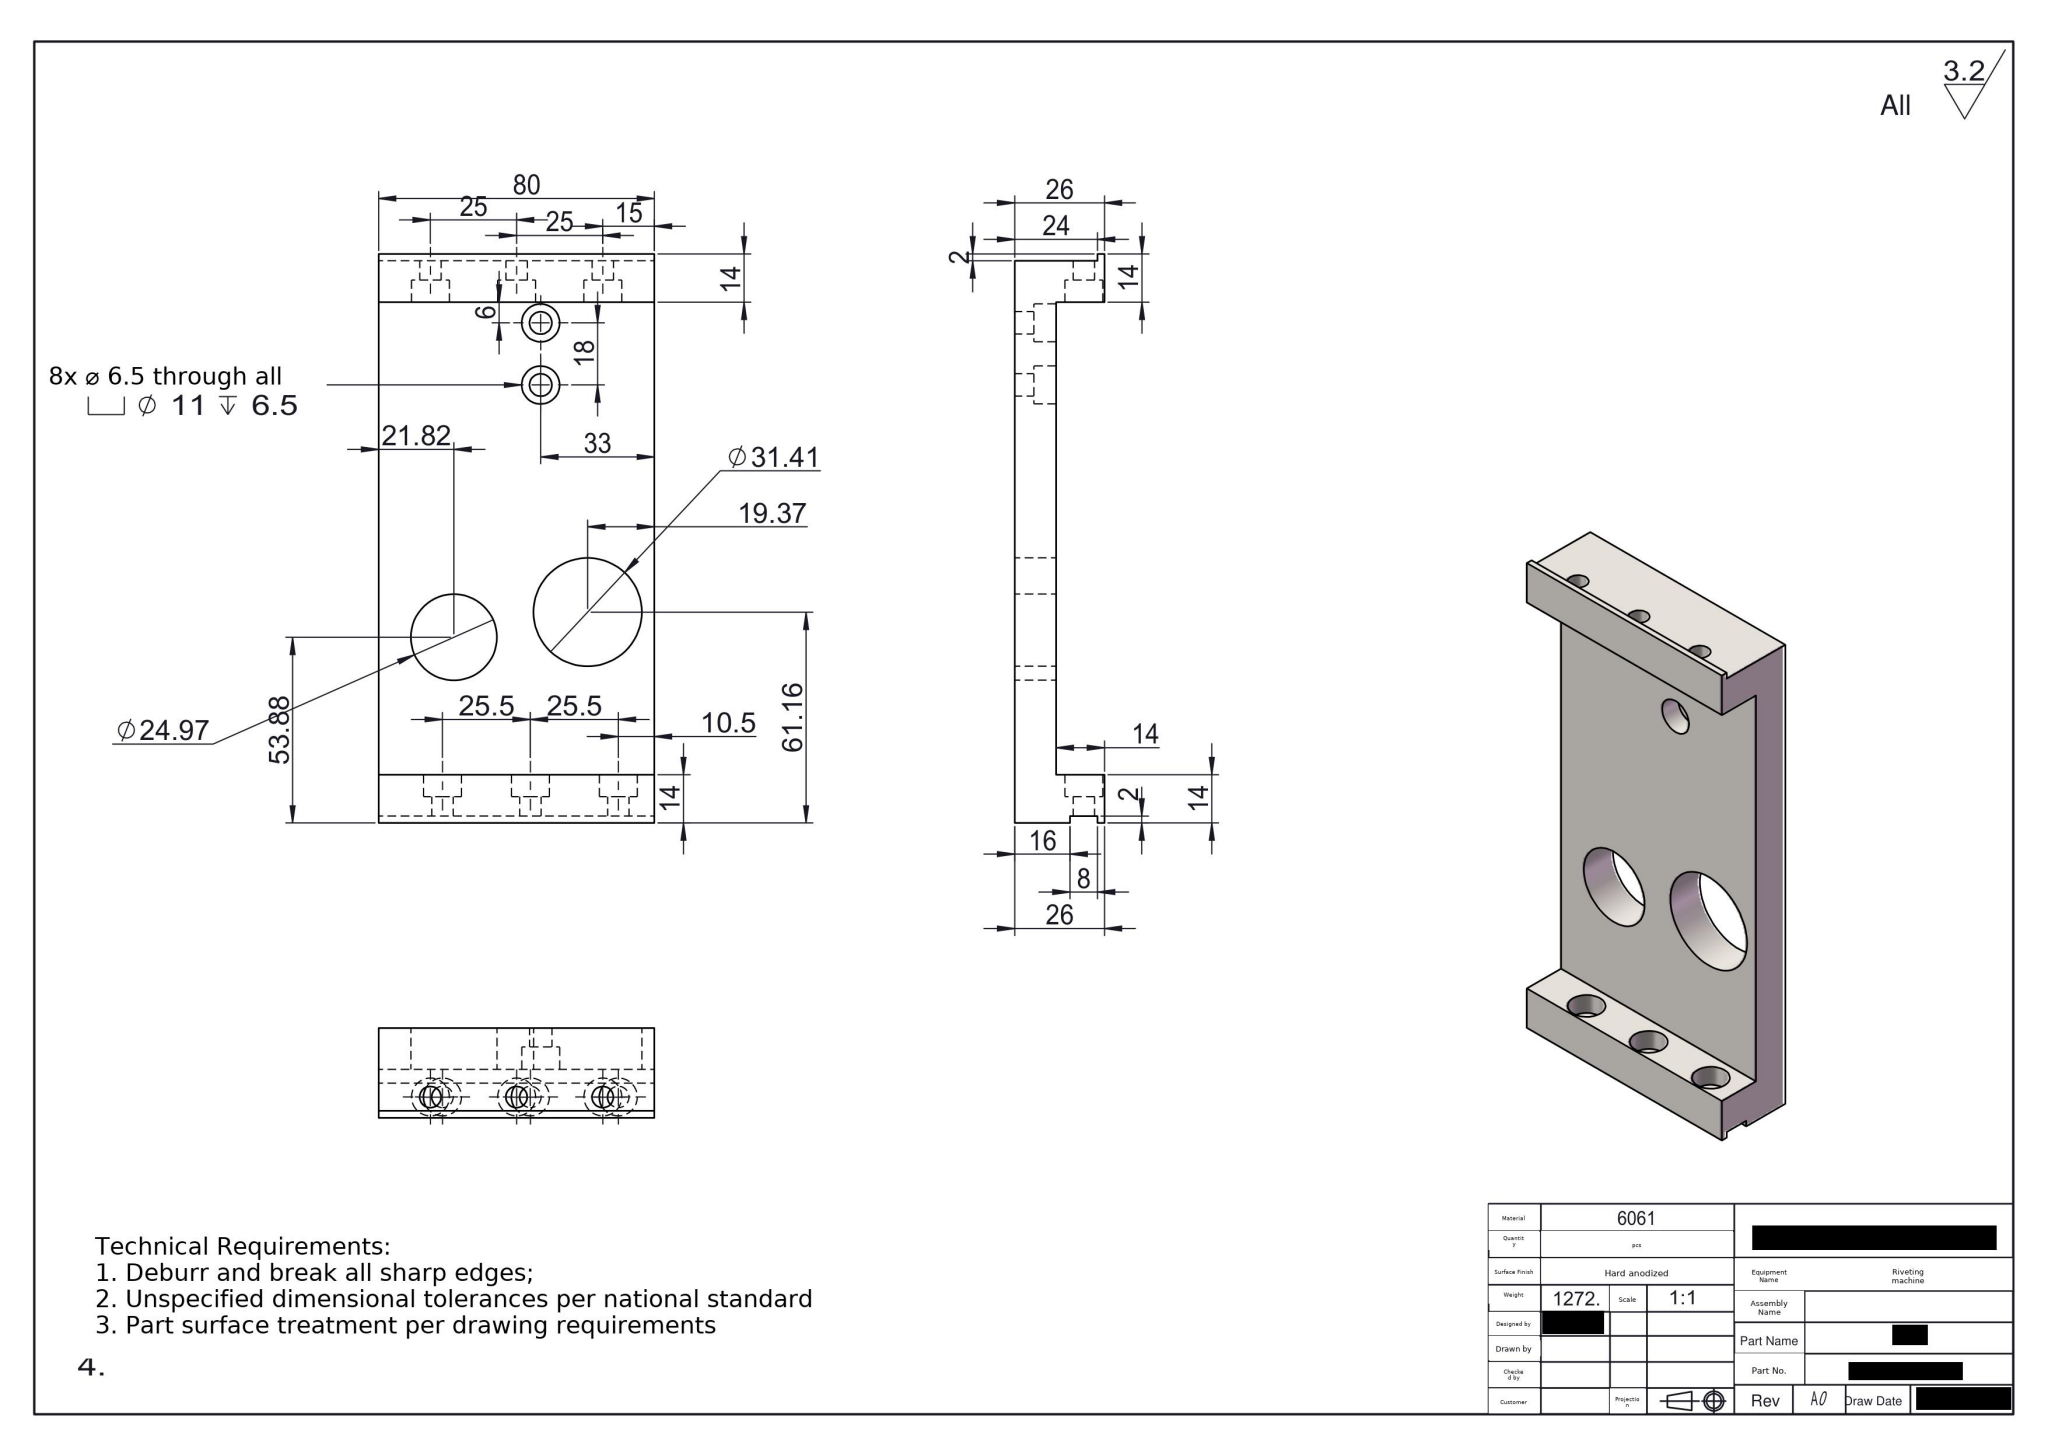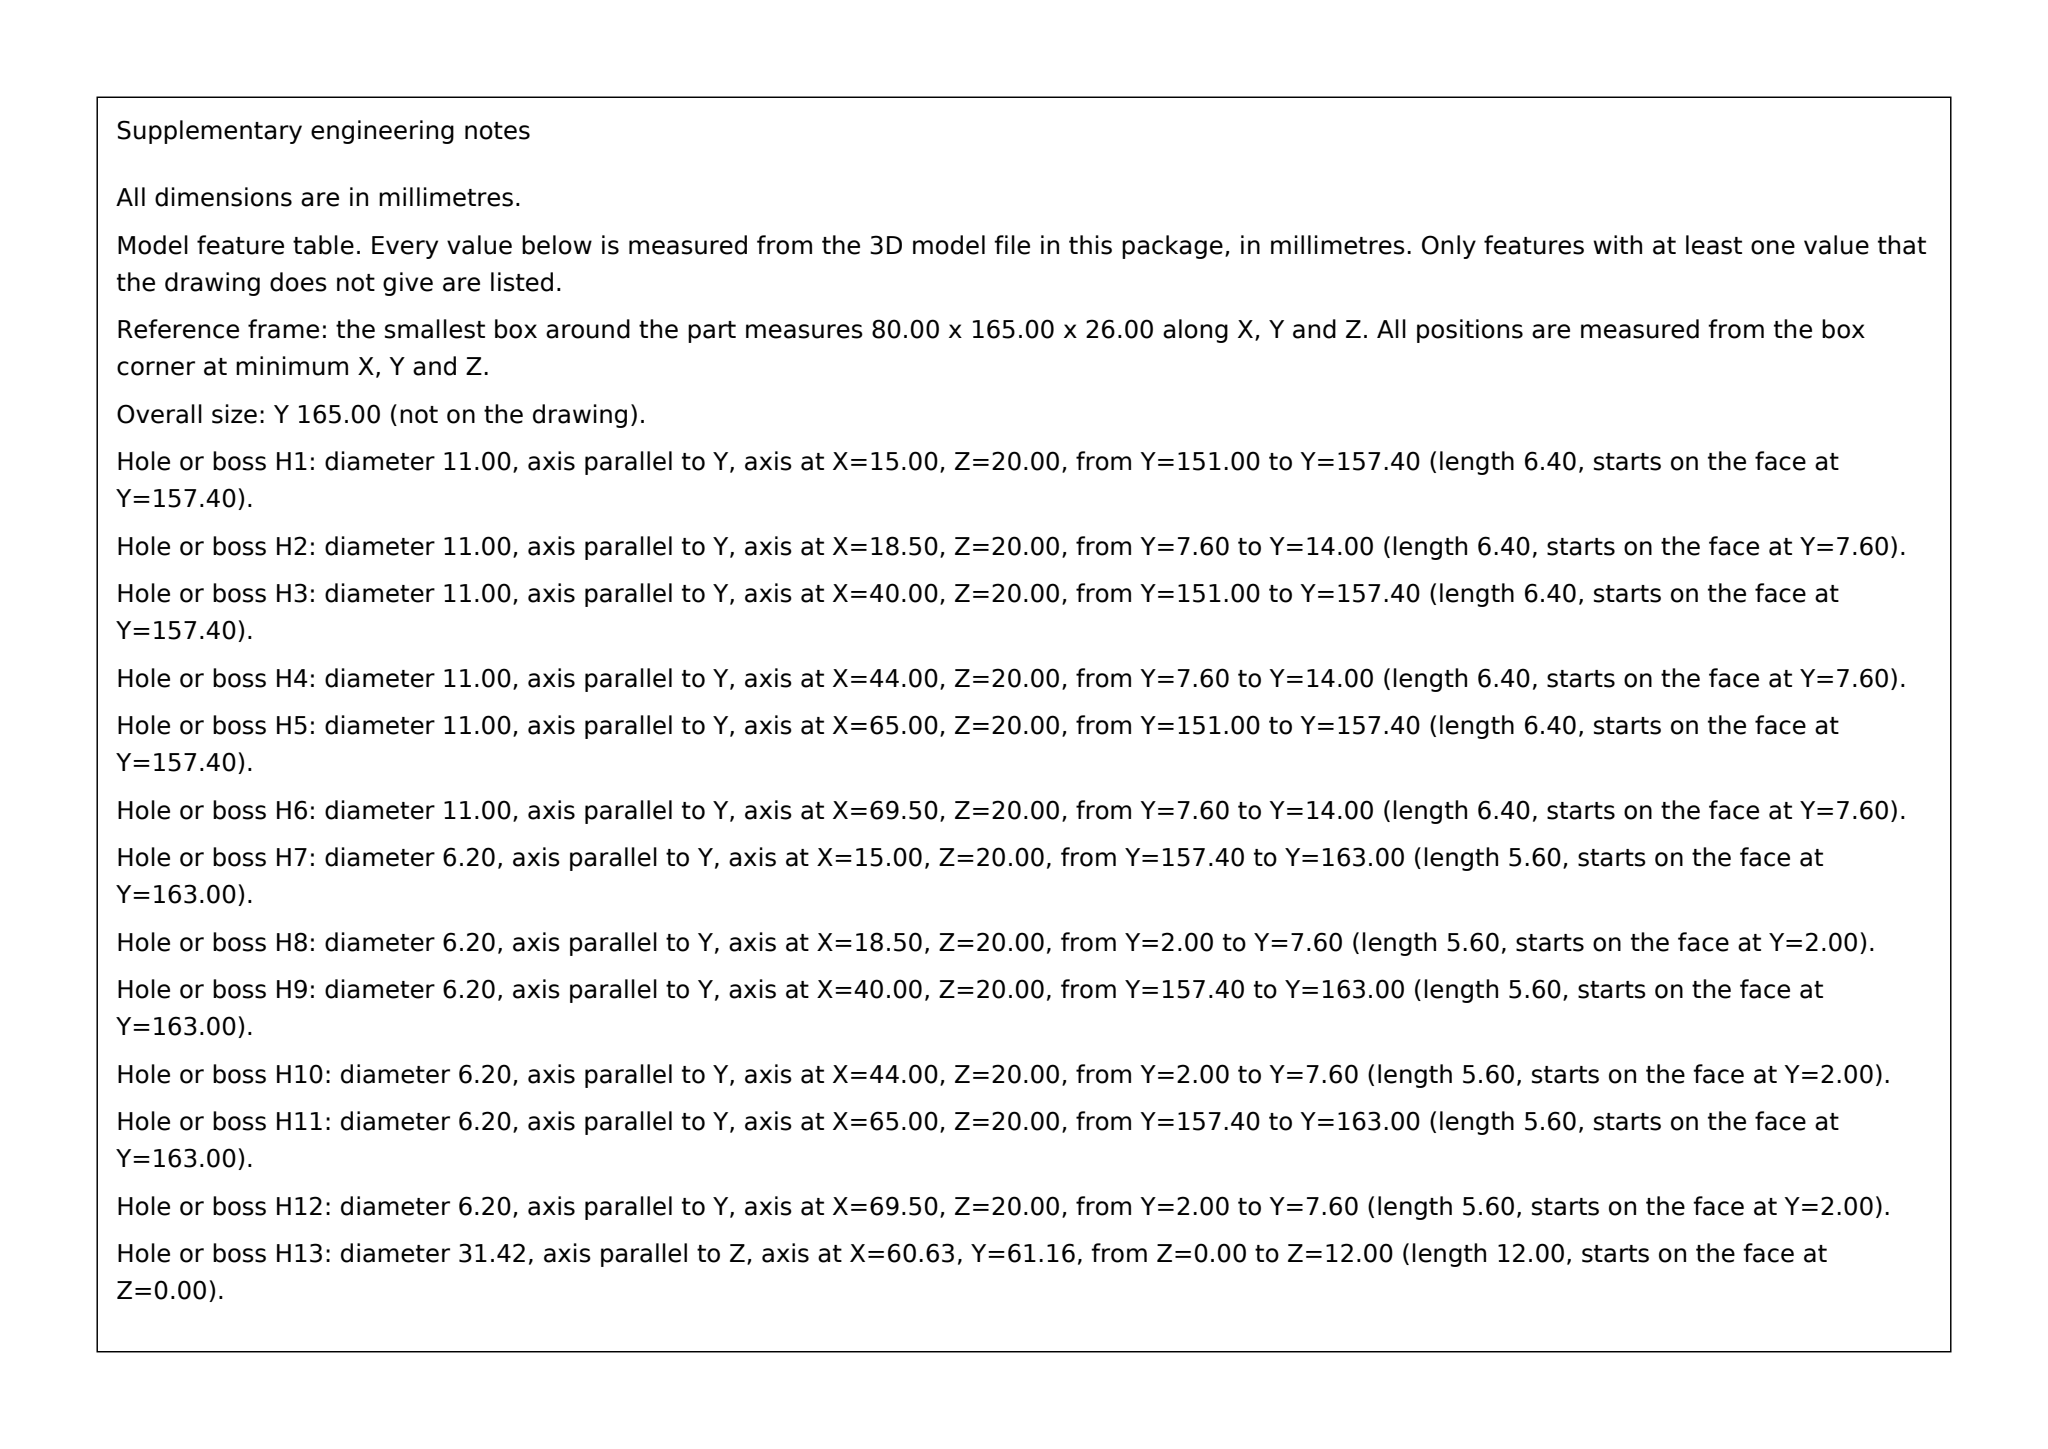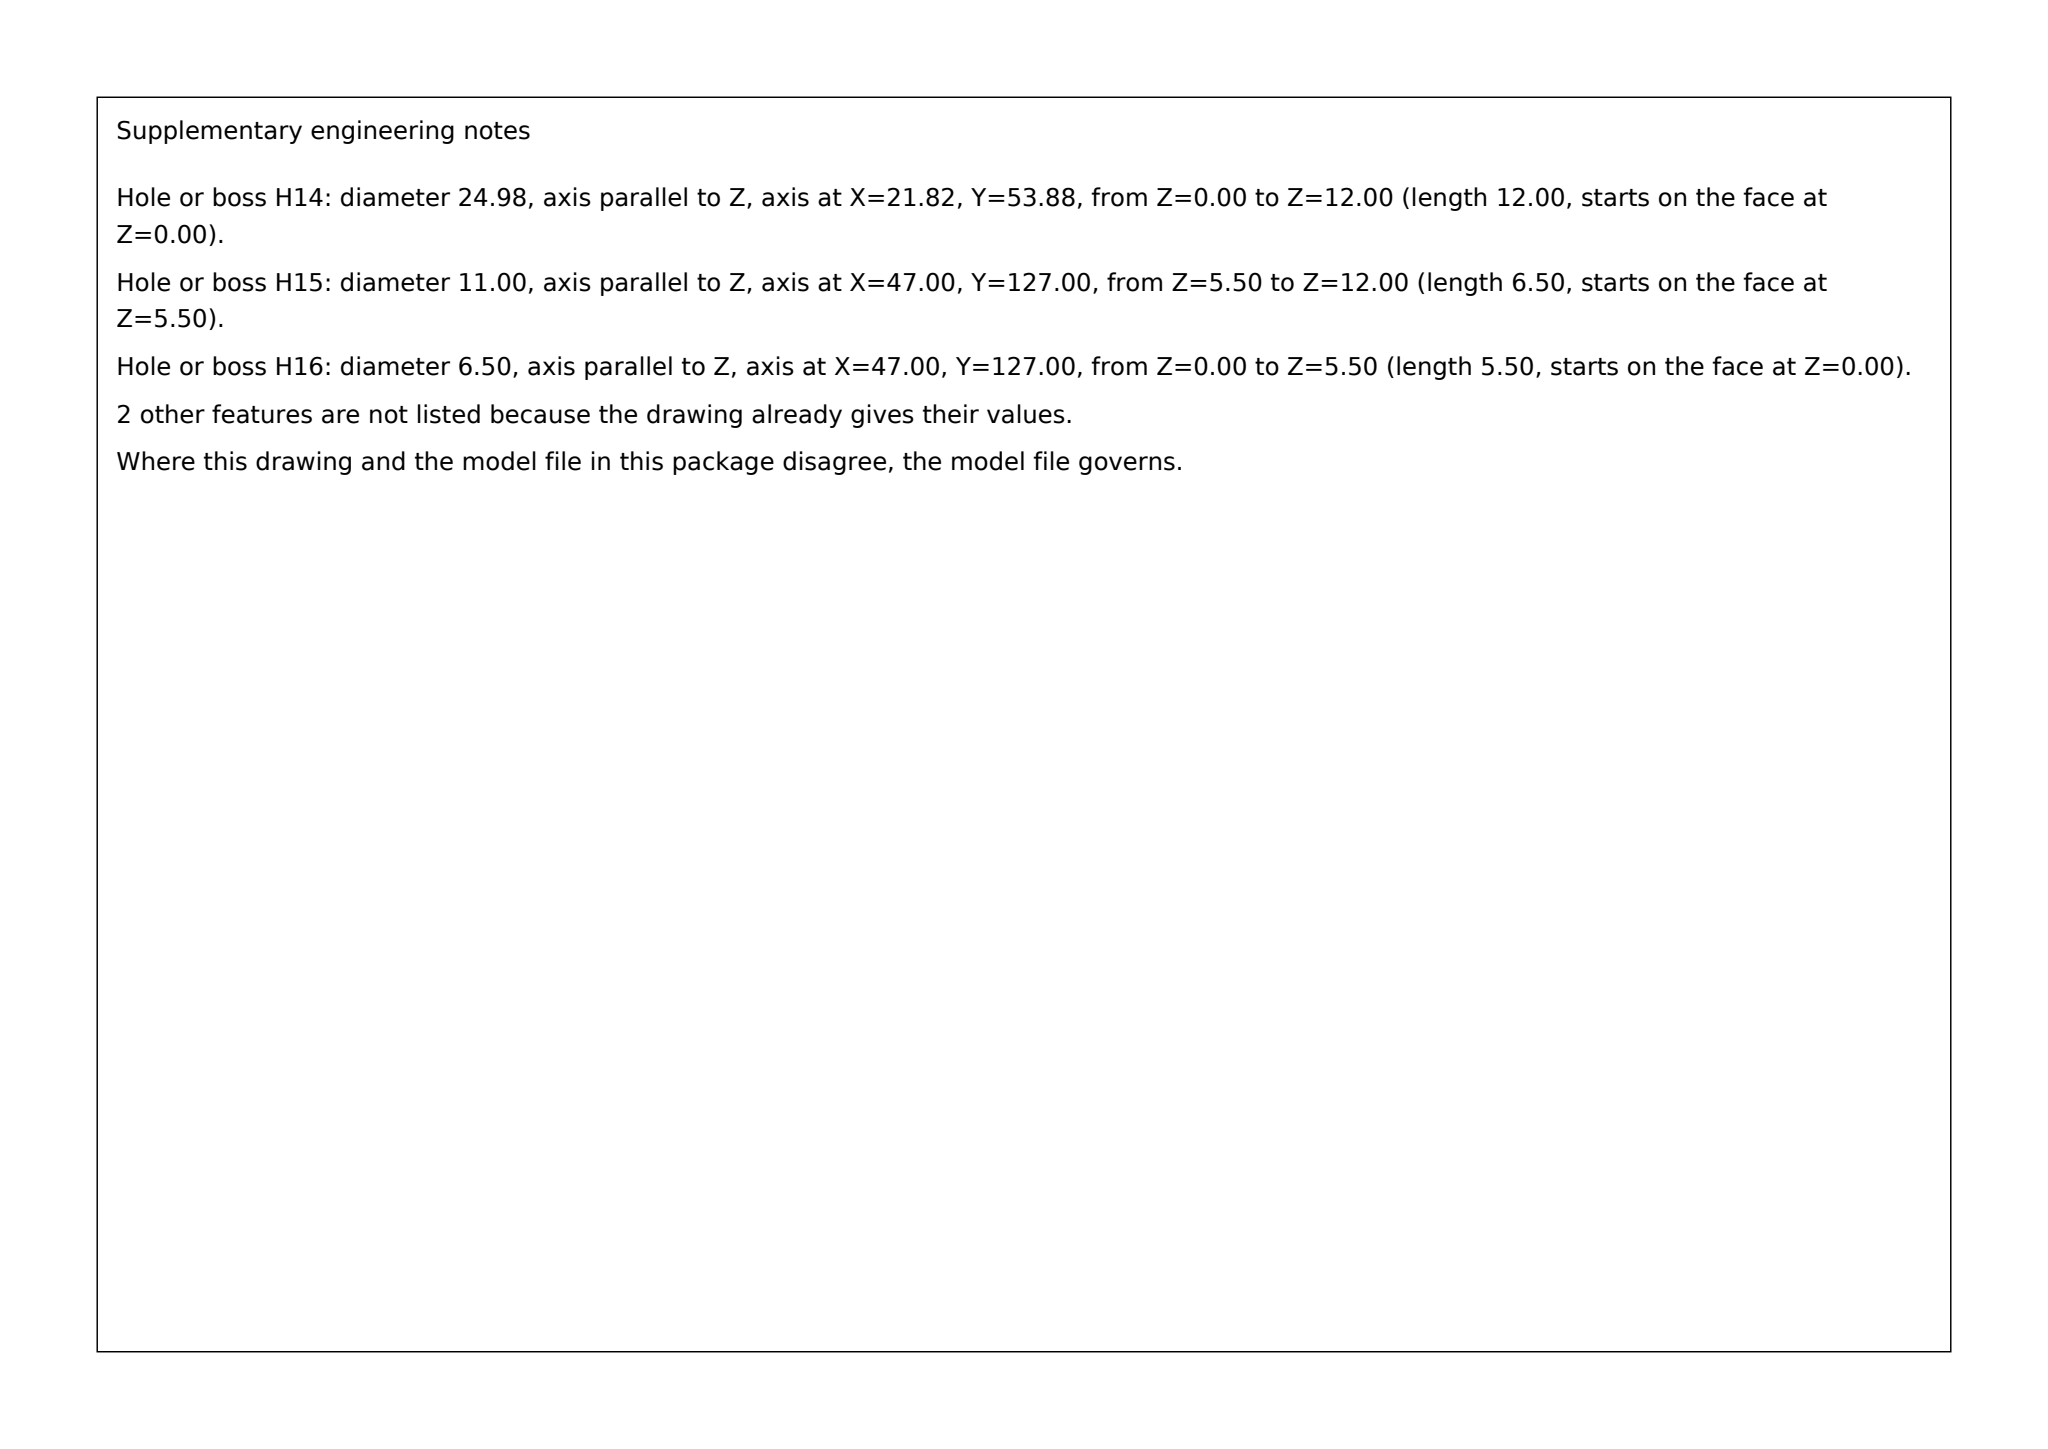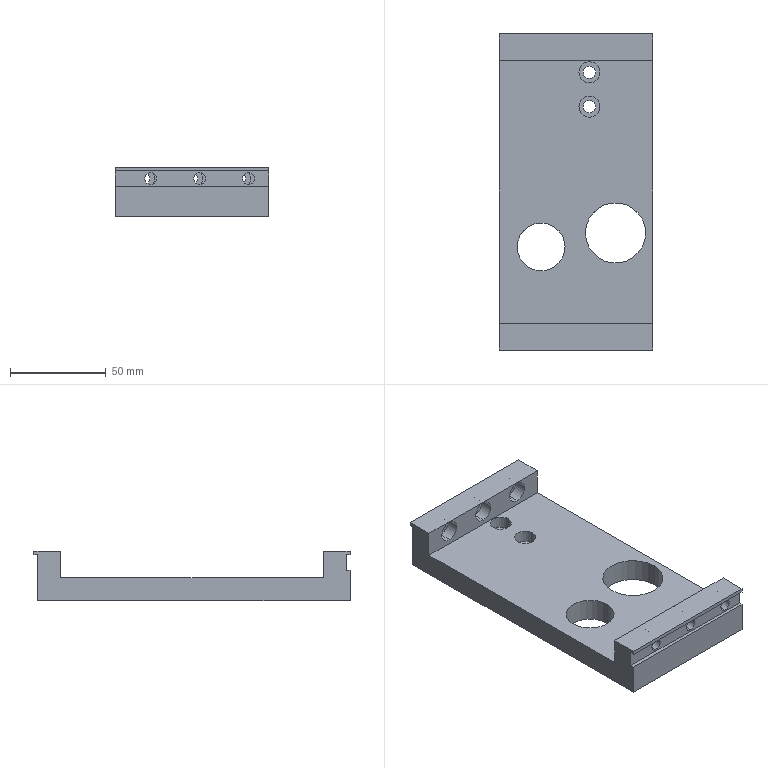Part | SolidWorks | mm | material 6061 | 1 solid | 60 faces | box 80 x 165 x 26 mm | volume 163198 mm3 | cylinder 36 | plane 24 | commonest cylinder face diameters 11 x16 6.2 x12 6.5 x4 24.971 x2 31.414 x2